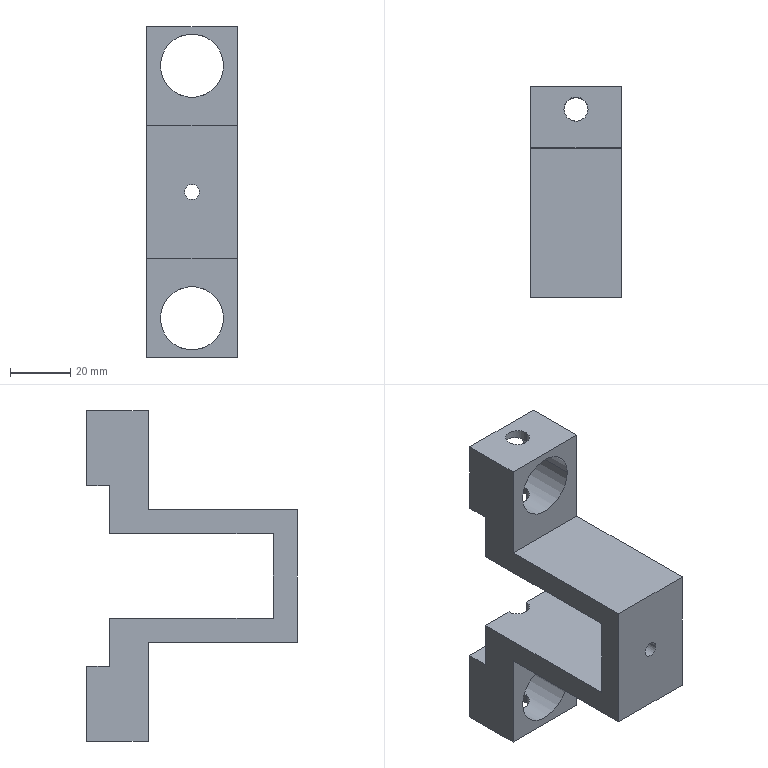Component | SolidWorks | JL001-05-03-1_JL001-05-01-007-1 | 1 solid | 50 faces | box 30 x 70 x 110 mm | volume 57621 mm3 | cylinder 22 | plane 20 | cone 8 | commonest cylinder face diameters 3.3 x8 8 x8 21 x4 5 x2
build123d program:
from build123d import *

# Parameters (mm, degrees)
SKETCH1_W                  = 110
SKETCH1_H                  = 70
BOSS_EXTRUDE1_DEPTH        = 15
F_21_0_21_DIAMETER_HOLE2_D = 21
SKETCH5_W                  = 33
SKETCH5_H                  = 49.6
SKETCH5_W_2                = 28
SKETCH5_H_2                = 124
CUT_EXTRUDE2_DEPTH         = 72.764
SIZE_MM_DOWEL_PIN_HOLE2_D  = 8
M6_TAPPED_HOLE1_D          = 5
SKETCH18_W                 = 60
SKETCH18_H                 = 7.5
CUT_EXTRUDE3_DEPTH         = 72.764
M4_TAPPED_HOLE1_D          = 3.3
M4_TAPPED_HOLE1_DEPTH      = 10.1
M4_TAPPED_HOLE1_TIP        = 0.9914


with BuildPart() as part:
    # Sketch1 → Boss-Extrude1 (new, symmetric)
    with BuildSketch(Plane.XY):
        Rectangle(SKETCH1_W, SKETCH1_H)
    extrude(amount=BOSS_EXTRUDE1_DEPTH, both=True)

    # 21.0 _21_ Diameter Hole2 (through all)
    with Locations(Plane(origin=(0, 35, 0), x_dir=(1, 0, 0), z_dir=(0, 1, 0))):
        with Locations((-42, 0), (42, 0)):
            Hole(F_21_0_21_DIAMETER_HOLE2_D / 2)

    # Sketch5 → Cut-Extrude2 (cut, through all)
    with BuildSketch(Plane.XY.offset(15)):
        with Locations((-38.5, -10.2)):
            Rectangle(SKETCH5_W, SKETCH5_H)
        with Locations((38.5, -10.2)):
            Rectangle(SKETCH5_W, SKETCH5_H)
        with Locations((0, 35)):
            Rectangle(SKETCH5_W_2, SKETCH5_H_2)
    extrude(amount=-CUT_EXTRUDE2_DEPTH, mode=Mode.SUBTRACT)

    # Size mm Dowel Pin Hole2 (through all)
    with Locations(Plane.ZY.offset(55)):
        with Locations((0, 27.5)):
            Hole(SIZE_MM_DOWEL_PIN_HOLE2_D / 2)

    # M6 Tapped Hole1 (through all)
    with Locations(Plane(origin=(0, -35, 0), x_dir=(-1, 0, 0), z_dir=(0, -1, 0))):
        with Locations((0, 0)):
            Hole(M6_TAPPED_HOLE1_D / 2)

    # Sketch18 → Cut-Extrude3 (cut, through all)
    with BuildSketch(Plane.XY.offset(15)):
        with Locations((0, 31.25)):
            Rectangle(SKETCH18_W, SKETCH18_H)
    extrude(amount=-CUT_EXTRUDE3_DEPTH, mode=Mode.SUBTRACT)

    # M4 Tapped Hole1
    with Locations(Plane(origin=(0, 27.5, 0), x_dir=(1, 0, 0), z_dir=(0, 1, 0))):
        with Locations((-22, -9), (-22, 9), (22, 9), (22, -9)):
            Hole(M4_TAPPED_HOLE1_D / 2, depth=M4_TAPPED_HOLE1_DEPTH)
            with Locations((0, 0, -(M4_TAPPED_HOLE1_DEPTH + M4_TAPPED_HOLE1_TIP / 2))):  # 118° drill point
                Cone(0, M4_TAPPED_HOLE1_D / 2, M4_TAPPED_HOLE1_TIP, mode=Mode.SUBTRACT)


solid = part.part

# Placed as in the assembly
solid = solid.moved(Location((0, 267.348, 63), (0, 90, 0)))